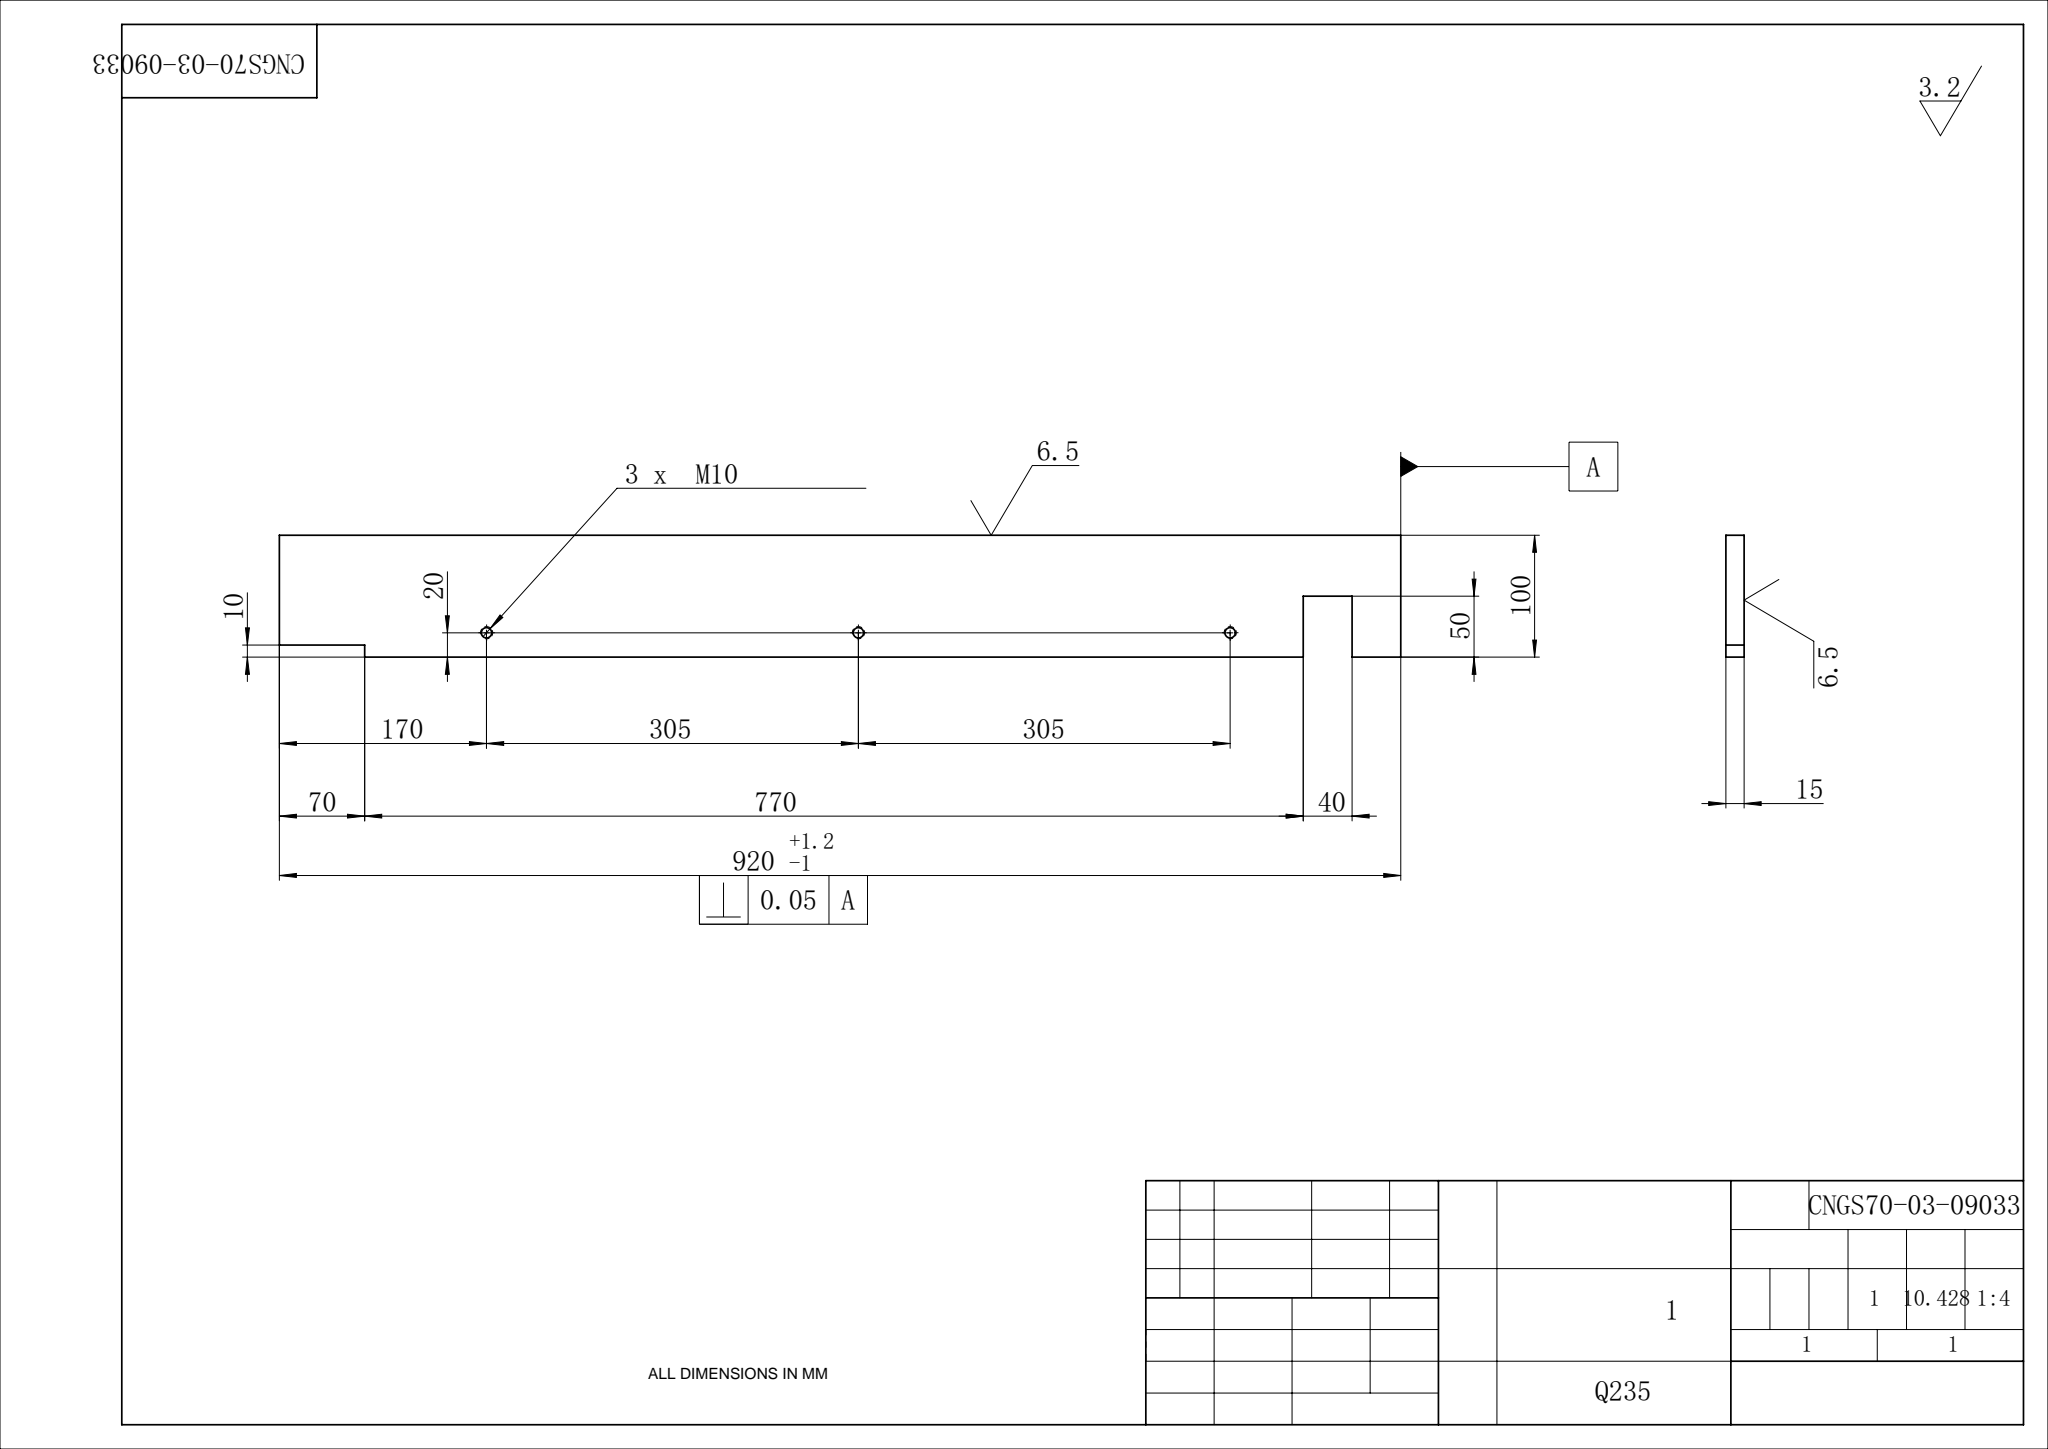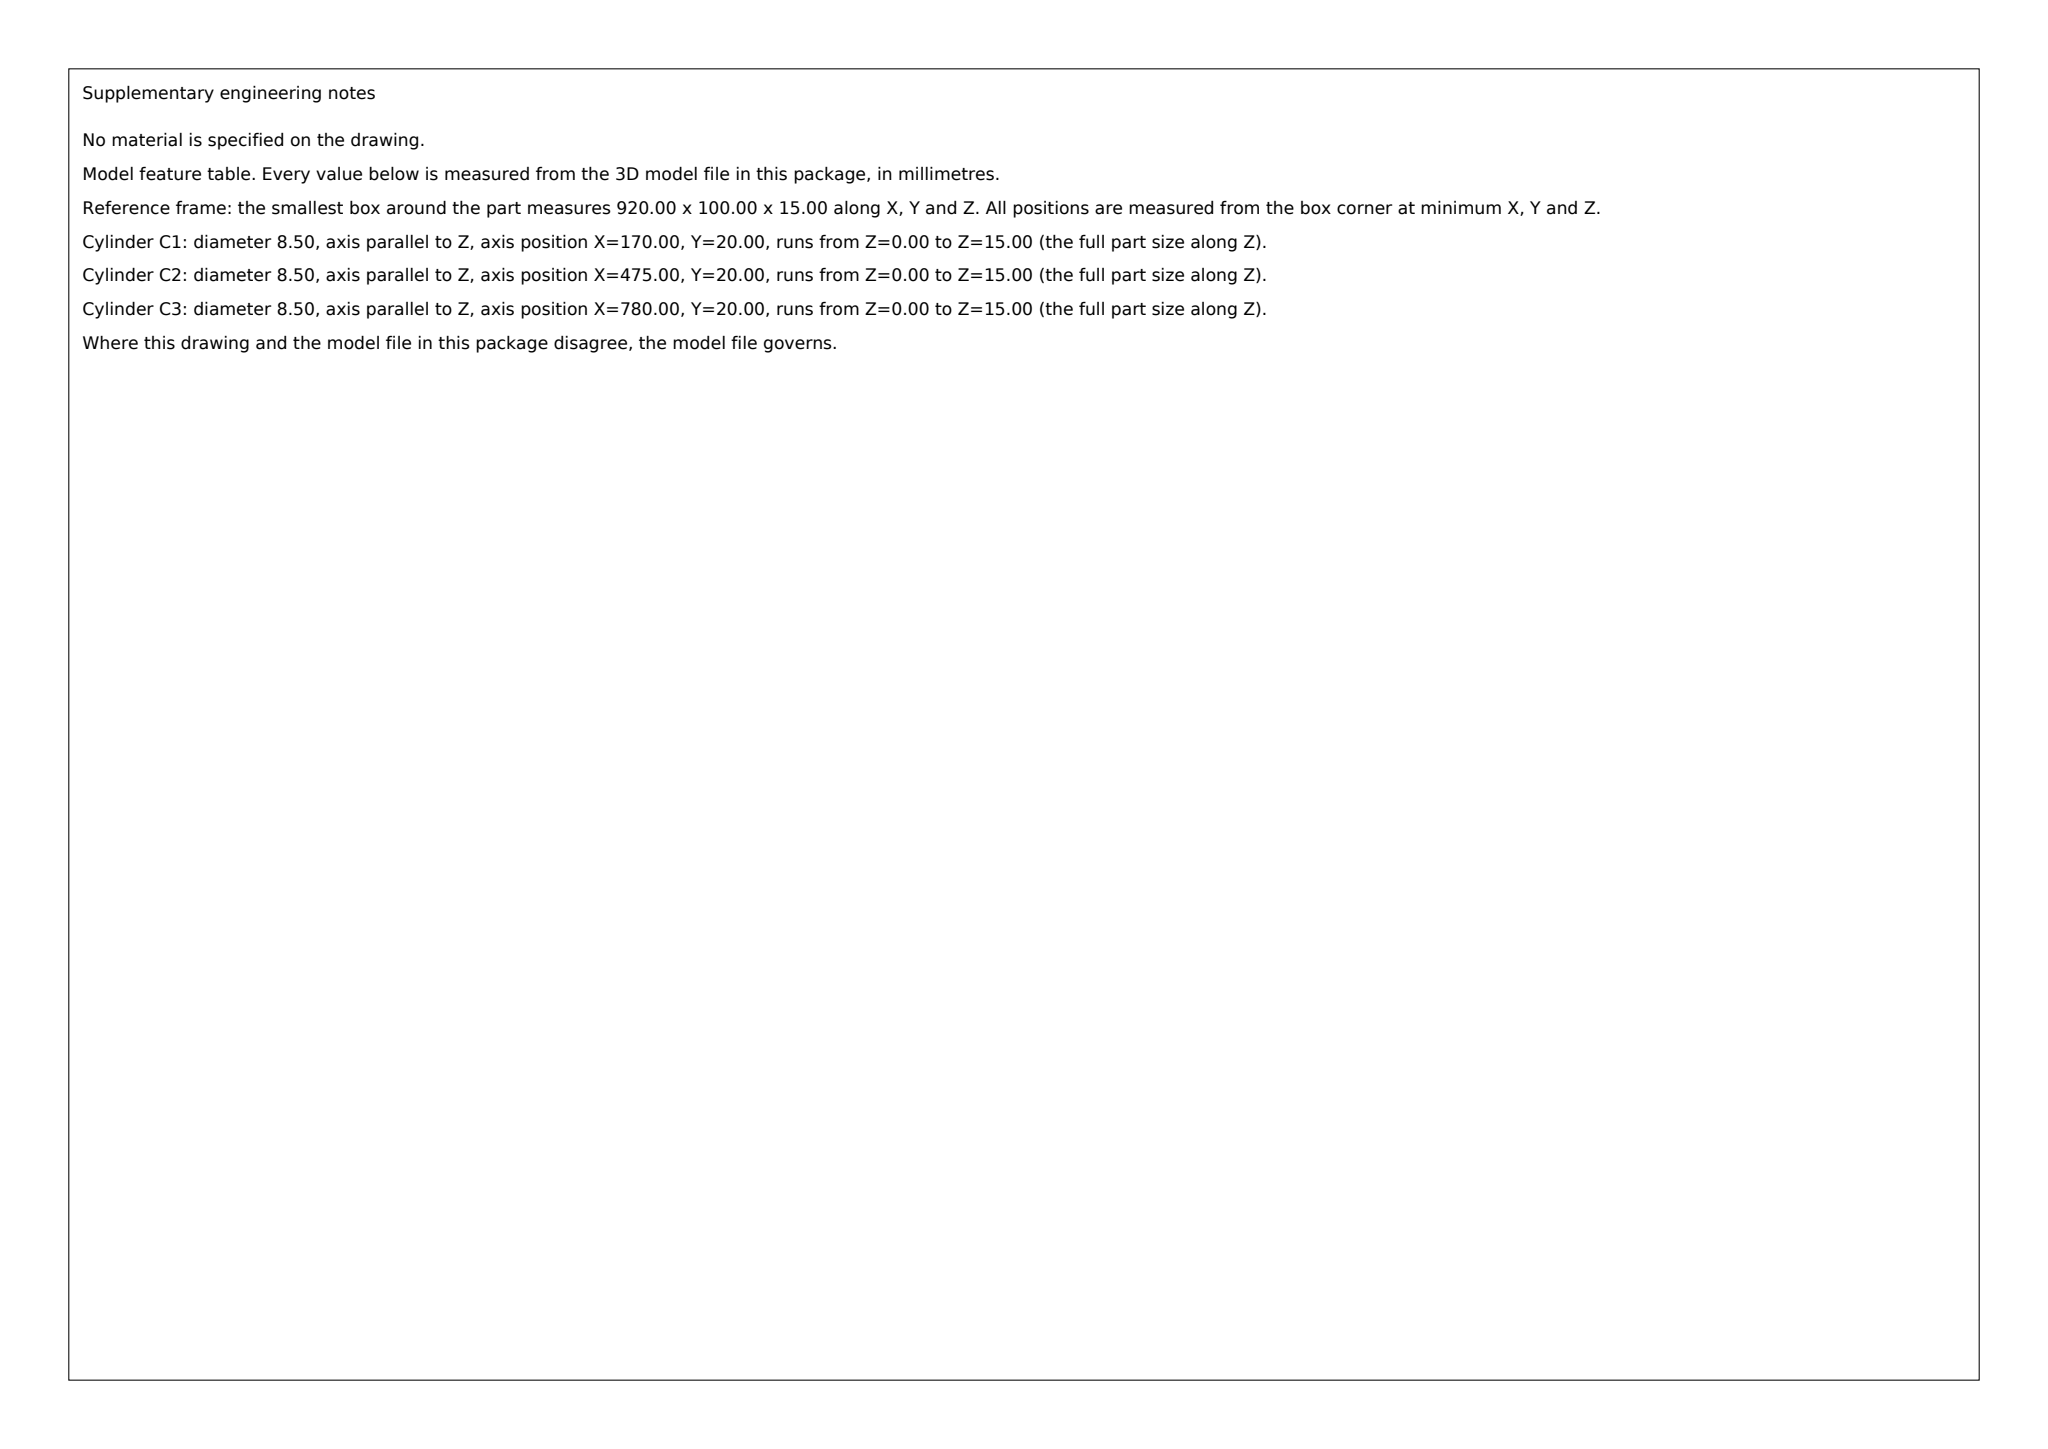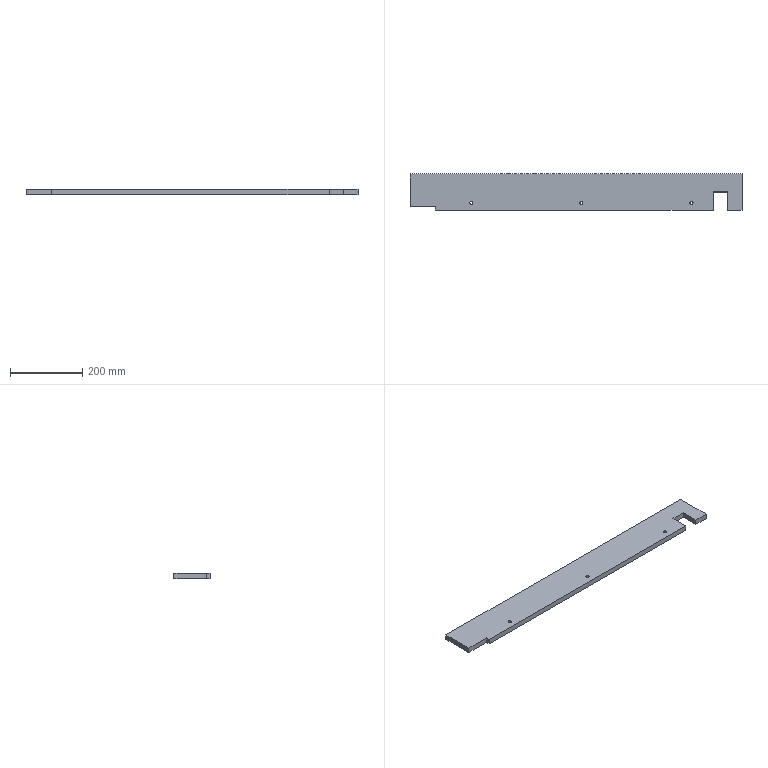Part | SolidWorks | mm | material Q235 | 1 solid | 18 faces | box 920 x 100 x 15 mm | volume 1336946 mm3 | plane 12 | cylinder 6 | commonest cylinder face diameters 8.5 x6
build123d program:
from build123d import *

# Parameters (mm, degrees)
SKETCH1_W              = 920
SKETCH1_H              = 100
BOSS_EXTRUDE1_DEPTH    = 15
M10_TAPPED_HOLE1_D     = 8.5
M10_TAPPED_HOLE1_DEPTH = 27.5
M10_TAPPED_HOLE1_TIP   = 2.554
SKETCH6_W              = 40
SKETCH6_H              = 50
SKETCH6_W_2            = 70
SKETCH6_H_2            = 10
CUT_EXTRUDE1_DEPTH     = 926.54


with BuildPart() as part:
    # Sketch1 → Boss-Extrude1 (new body)
    with BuildSketch(Plane.XY):
        with Locations((460, 50)):
            Rectangle(SKETCH1_W, SKETCH1_H)
    extrude(amount=BOSS_EXTRUDE1_DEPTH)

    # M10 Tapped Hole1
    with Locations(Plane(origin=(0, 0, 0), x_dir=(-1, 0, 0), z_dir=(0, 0, -1))):
        with Locations((-780, 20), (-475, 20), (-170, 20)):
            Hole(M10_TAPPED_HOLE1_D / 2, depth=M10_TAPPED_HOLE1_DEPTH)
            with Locations((0, 0, -(M10_TAPPED_HOLE1_DEPTH + M10_TAPPED_HOLE1_TIP / 2))):  # 118° drill point
                Cone(0, M10_TAPPED_HOLE1_D / 2, M10_TAPPED_HOLE1_TIP, mode=Mode.SUBTRACT)

    # Sketch6 → Cut-Extrude1 (cut, through all)
    with BuildSketch(Plane.XY.offset(15)):
        with Locations((860, 25)):
            Rectangle(SKETCH6_W, SKETCH6_H)
        with Locations((35, 5)):
            Rectangle(SKETCH6_W_2, SKETCH6_H_2)
    extrude(amount=-CUT_EXTRUDE1_DEPTH, mode=Mode.SUBTRACT)


solid = part.part
STEP:
#1=CARTESIAN_POINT('',(775.75,20.,15.));
#2=VERTEX_POINT('',#1);
#3=CARTESIAN_POINT('',(784.25,20.,15.));
#4=VERTEX_POINT('',#3);
#5=CARTESIAN_POINT('',(780.,20.,15.));
#6=DIRECTION('',(0.,0.,1.));
#7=DIRECTION('',(1.,0.,0.));
#8=AXIS2_PLACEMENT_3D('',#5,#6,#7);
#9=CIRCLE('',#8,4.25);
#10=EDGE_CURVE('',#2,#4,#9,.T.);
#11=ORIENTED_EDGE('',*,*,#10,.T.);
#12=CARTESIAN_POINT('',(784.25,20.,0.));
#13=VERTEX_POINT('',#12);
#14=CARTESIAN_POINT('',(784.25,20.,0.));
#15=DIRECTION('',(0.,0.,-1.));
#16=VECTOR('',#15,1000.);
#17=LINE('',#14,#16);
#18=EDGE_CURVE('',#4,#13,#17,.T.);
#19=ORIENTED_EDGE('',*,*,#18,.T.);
#20=CARTESIAN_POINT('',(775.75,20.,0.));
#21=VERTEX_POINT('',#20);
#22=CARTESIAN_POINT('',(780.,20.,0.));
#23=DIRECTION('',(0.,0.,-1.));
#24=DIRECTION('',(-1.,0.,0.));
#25=AXIS2_PLACEMENT_3D('',#22,#23,#24);
#26=CIRCLE('',#25,4.25);
#27=EDGE_CURVE('',#13,#21,#26,.T.);
#28=ORIENTED_EDGE('',*,*,#27,.T.);
#29=CARTESIAN_POINT('',(775.75,20.,0.));
#30=DIRECTION('',(0.,0.,-1.));
#31=VECTOR('',#30,1000.);
#32=LINE('',#29,#31);
#33=EDGE_CURVE('',#2,#21,#32,.T.);
#34=ORIENTED_EDGE('',*,*,#33,.F.);
#35=EDGE_LOOP('',(#11,#19,#28,#34));
#36=FACE_OUTER_BOUND('',#35,.T.);
#37=CARTESIAN_POINT('',(780.,20.,0.));
#38=DIRECTION('',(0.,0.,-1.));
#39=DIRECTION('',(-1.,0.,0.));
#40=AXIS2_PLACEMENT_3D('',#37,#38,#39);
#41=CYLINDRICAL_SURFACE('',#40,4.25);
#42=ADVANCED_FACE('',(#36),#41,.F.);
#43=CARTESIAN_POINT('',(470.75,20.,15.));
#44=VERTEX_POINT('',#43);
#45=CARTESIAN_POINT('',(479.25,20.,15.));
#46=VERTEX_POINT('',#45);
#47=CARTESIAN_POINT('',(475.,20.,15.));
#48=DIRECTION('',(0.,0.,1.));
#49=DIRECTION('',(1.,0.,0.));
#50=AXIS2_PLACEMENT_3D('',#47,#48,#49);
#51=CIRCLE('',#50,4.25);
#52=EDGE_CURVE('',#44,#46,#51,.T.);
#53=ORIENTED_EDGE('',*,*,#52,.T.);
#54=CARTESIAN_POINT('',(479.25,20.,0.));
#55=VERTEX_POINT('',#54);
#56=CARTESIAN_POINT('',(479.25,20.,0.));
#57=DIRECTION('',(0.,0.,-1.));
#58=VECTOR('',#57,1000.);
#59=LINE('',#56,#58);
#60=EDGE_CURVE('',#46,#55,#59,.T.);
#61=ORIENTED_EDGE('',*,*,#60,.T.);
#62=CARTESIAN_POINT('',(470.75,20.,0.));
#63=VERTEX_POINT('',#62);
#64=CARTESIAN_POINT('',(475.,20.,0.));
#65=DIRECTION('',(0.,0.,-1.));
#66=DIRECTION('',(-1.,0.,0.));
#67=AXIS2_PLACEMENT_3D('',#64,#65,#66);
#68=CIRCLE('',#67,4.25);
#69=EDGE_CURVE('',#55,#63,#68,.T.);
#70=ORIENTED_EDGE('',*,*,#69,.T.);
#71=CARTESIAN_POINT('',(470.75,20.,0.));
#72=DIRECTION('',(0.,0.,-1.));
#73=VECTOR('',#72,1000.);
#74=LINE('',#71,#73);
#75=EDGE_CURVE('',#44,#63,#74,.T.);
#76=ORIENTED_EDGE('',*,*,#75,.F.);
#77=EDGE_LOOP('',(#53,#61,#70,#76));
#78=FACE_OUTER_BOUND('',#77,.T.);
#79=CARTESIAN_POINT('',(475.,20.,0.));
#80=DIRECTION('',(0.,0.,-1.));
#81=DIRECTION('',(-1.,0.,0.));
#82=AXIS2_PLACEMENT_3D('',#79,#80,#81);
#83=CYLINDRICAL_SURFACE('',#82,4.25);
#84=ADVANCED_FACE('',(#78),#83,.F.);
#85=CARTESIAN_POINT('',(165.75,20.,15.));
#86=VERTEX_POINT('',#85);
#87=CARTESIAN_POINT('',(174.25,20.,15.));
#88=VERTEX_POINT('',#87);
#89=CARTESIAN_POINT('',(170.,20.,15.));
#90=DIRECTION('',(0.,0.,1.));
#91=DIRECTION('',(1.,0.,0.));
#92=AXIS2_PLACEMENT_3D('',#89,#90,#91);
#93=CIRCLE('',#92,4.25);
#94=EDGE_CURVE('',#86,#88,#93,.T.);
#95=ORIENTED_EDGE('',*,*,#94,.T.);
#96=CARTESIAN_POINT('',(174.25,20.,0.));
#97=VERTEX_POINT('',#96);
#98=CARTESIAN_POINT('',(174.25,20.,0.));
#99=DIRECTION('',(0.,0.,-1.));
#100=VECTOR('',#99,1000.);
#101=LINE('',#98,#100);
#102=EDGE_CURVE('',#88,#97,#101,.T.);
#103=ORIENTED_EDGE('',*,*,#102,.T.);
#104=CARTESIAN_POINT('',(165.75,20.,0.));
#105=VERTEX_POINT('',#104);
#106=CARTESIAN_POINT('',(170.,20.,0.));
#107=DIRECTION('',(0.,0.,-1.));
#108=DIRECTION('',(-1.,0.,0.));
#109=AXIS2_PLACEMENT_3D('',#106,#107,#108);
#110=CIRCLE('',#109,4.25);
#111=EDGE_CURVE('',#97,#105,#110,.T.);
#112=ORIENTED_EDGE('',*,*,#111,.T.);
#113=CARTESIAN_POINT('',(165.75,20.,0.));
#114=DIRECTION('',(0.,0.,-1.));
#115=VECTOR('',#114,1000.);
#116=LINE('',#113,#115);
#117=EDGE_CURVE('',#86,#105,#116,.T.);
#118=ORIENTED_EDGE('',*,*,#117,.F.);
#119=EDGE_LOOP('',(#95,#103,#112,#118));
#120=FACE_OUTER_BOUND('',#119,.T.);
#121=CARTESIAN_POINT('',(170.,20.,0.));
#122=DIRECTION('',(0.,0.,-1.));
#123=DIRECTION('',(-1.,0.,0.));
#124=AXIS2_PLACEMENT_3D('',#121,#122,#123);
#125=CYLINDRICAL_SURFACE('',#124,4.25);
#126=ADVANCED_FACE('',(#120),#125,.F.);
#127=CARTESIAN_POINT('',(70.,0.,15.));
#128=VERTEX_POINT('',#127);
#129=CARTESIAN_POINT('',(840.,0.,15.));
#130=VERTEX_POINT('',#129);
#131=CARTESIAN_POINT('',(0.,0.,15.));
#132=DIRECTION('',(1.,0.,0.));
#133=VECTOR('',#132,1000.);
#134=LINE('',#131,#133);
#135=EDGE_CURVE('',#128,#130,#134,.T.);
#136=ORIENTED_EDGE('',*,*,#135,.F.);
#137=CARTESIAN_POINT('',(70.,0.,0.));
#138=VERTEX_POINT('',#137);
#139=CARTESIAN_POINT('',(70.,0.,0.));
#140=DIRECTION('',(0.,0.,1.));
#141=VECTOR('',#140,1000.);
#142=LINE('',#139,#141);
#143=EDGE_CURVE('',#138,#128,#142,.T.);
#144=ORIENTED_EDGE('',*,*,#143,.F.);
#145=CARTESIAN_POINT('',(840.,0.,0.));
#146=VERTEX_POINT('',#145);
#147=CARTESIAN_POINT('',(0.,0.,0.));
#148=DIRECTION('',(1.,0.,0.));
#149=VECTOR('',#148,1000.);
#150=LINE('',#147,#149);
#151=EDGE_CURVE('',#138,#146,#150,.T.);
#152=ORIENTED_EDGE('',*,*,#151,.T.);
#153=CARTESIAN_POINT('',(840.,0.,0.));
#154=DIRECTION('',(0.,0.,1.));
#155=VECTOR('',#154,1000.);
#156=LINE('',#153,#155);
#157=EDGE_CURVE('',#146,#130,#156,.T.);
#158=ORIENTED_EDGE('',*,*,#157,.T.);
#159=EDGE_LOOP('',(#136,#144,#152,#158));
#160=FACE_OUTER_BOUND('',#159,.T.);
#161=CARTESIAN_POINT('',(0.,0.,15.));
#162=DIRECTION('',(0.,1.,0.));
#163=DIRECTION('',(0.,0.,1.));
#164=AXIS2_PLACEMENT_3D('',#161,#162,#163);
#165=PLANE('',#164);
#166=ADVANCED_FACE('',(#160),#165,.F.);
#167=CARTESIAN_POINT('',(920.,100.,0.));
#168=VERTEX_POINT('',#167);
#169=CARTESIAN_POINT('',(920.,0.,0.));
#170=VERTEX_POINT('',#169);
#171=CARTESIAN_POINT('',(920.,0.,0.));
#172=DIRECTION('',(0.,-1.,0.));
#173=VECTOR('',#172,1000.);
#174=LINE('',#171,#173);
#175=EDGE_CURVE('',#168,#170,#174,.T.);
#176=ORIENTED_EDGE('',*,*,#175,.F.);
#177=CARTESIAN_POINT('',(920.,100.,15.));
#178=VERTEX_POINT('',#177);
#179=CARTESIAN_POINT('',(920.,100.,15.));
#180=DIRECTION('',(0.,0.,-1.));
#181=VECTOR('',#180,1000.);
#182=LINE('',#179,#181);
#183=EDGE_CURVE('',#178,#168,#182,.T.);
#184=ORIENTED_EDGE('',*,*,#183,.F.);
#185=CARTESIAN_POINT('',(920.,0.,15.));
#186=VERTEX_POINT('',#185);
#187=CARTESIAN_POINT('',(920.,0.,15.));
#188=DIRECTION('',(0.,-1.,0.));
#189=VECTOR('',#188,1000.);
#190=LINE('',#187,#189);
#191=EDGE_CURVE('',#178,#186,#190,.T.);
#192=ORIENTED_EDGE('',*,*,#191,.T.);
#193=CARTESIAN_POINT('',(920.,0.,15.));
#194=DIRECTION('',(0.,0.,-1.));
#195=VECTOR('',#194,1000.);
#196=LINE('',#193,#195);
#197=EDGE_CURVE('',#186,#170,#196,.T.);
#198=ORIENTED_EDGE('',*,*,#197,.T.);
#199=EDGE_LOOP('',(#176,#184,#192,#198));
#200=FACE_OUTER_BOUND('',#199,.T.);
#201=CARTESIAN_POINT('',(920.,0.,15.));
#202=DIRECTION('',(1.,0.,0.));
#203=DIRECTION('',(0.,0.,-1.));
#204=AXIS2_PLACEMENT_3D('',#201,#202,#203);
#205=PLANE('',#204);
#206=ADVANCED_FACE('',(#200),#205,.T.);
#207=CARTESIAN_POINT('',(0.,100.,0.));
#208=VERTEX_POINT('',#207);
#209=CARTESIAN_POINT('',(0.,100.,0.));
#210=DIRECTION('',(1.,-0.,0.));
#211=VECTOR('',#210,1000.);
#212=LINE('',#209,#211);
#213=EDGE_CURVE('',#208,#168,#212,.T.);
#214=ORIENTED_EDGE('',*,*,#213,.F.);
#215=CARTESIAN_POINT('',(0.,100.,15.));
#216=VERTEX_POINT('',#215);
#217=CARTESIAN_POINT('',(0.,100.,15.));
#218=DIRECTION('',(0.,0.,-1.));
#219=VECTOR('',#218,1000.);
#220=LINE('',#217,#219);
#221=EDGE_CURVE('',#216,#208,#220,.T.);
#222=ORIENTED_EDGE('',*,*,#221,.F.);
#223=CARTESIAN_POINT('',(0.,100.,15.));
#224=DIRECTION('',(1.,-0.,0.));
#225=VECTOR('',#224,1000.);
#226=LINE('',#223,#225);
#227=EDGE_CURVE('',#216,#178,#226,.T.);
#228=ORIENTED_EDGE('',*,*,#227,.T.);
#229=ORIENTED_EDGE('',*,*,#183,.T.);
#230=EDGE_LOOP('',(#214,#222,#228,#229));
#231=FACE_OUTER_BOUND('',#230,.T.);
#232=CARTESIAN_POINT('',(0.,100.,15.));
#233=DIRECTION('',(0.,1.,0.));
#234=DIRECTION('',(-1.,0.,0.));
#235=AXIS2_PLACEMENT_3D('',#232,#233,#234);
#236=PLANE('',#235);
#237=ADVANCED_FACE('',(#231),#236,.T.);
#238=CARTESIAN_POINT('',(0.,10.,0.));
#239=VERTEX_POINT('',#238);
#240=CARTESIAN_POINT('',(0.,10.,15.));
#241=VERTEX_POINT('',#240);
#242=CARTESIAN_POINT('',(0.,10.,0.));
#243=DIRECTION('',(0.,0.,1.));
#244=VECTOR('',#243,1000.);
#245=LINE('',#242,#244);
#246=EDGE_CURVE('',#239,#241,#245,.T.);
#247=ORIENTED_EDGE('',*,*,#246,.T.);
#248=CARTESIAN_POINT('',(0.,0.,15.));
#249=DIRECTION('',(0.,1.,0.));
#250=VECTOR('',#249,1000.);
#251=LINE('',#248,#250);
#252=EDGE_CURVE('',#241,#216,#251,.T.);
#253=ORIENTED_EDGE('',*,*,#252,.T.);
#254=ORIENTED_EDGE('',*,*,#221,.T.);
#255=CARTESIAN_POINT('',(0.,0.,0.));
#256=DIRECTION('',(0.,1.,0.));
#257=VECTOR('',#256,1000.);
#258=LINE('',#255,#257);
#259=EDGE_CURVE('',#239,#208,#258,.T.);
#260=ORIENTED_EDGE('',*,*,#259,.F.);
#261=EDGE_LOOP('',(#247,#253,#254,#260));
#262=FACE_OUTER_BOUND('',#261,.T.);
#263=CARTESIAN_POINT('',(0.,0.,15.));
#264=DIRECTION('',(-1.,0.,0.));
#265=DIRECTION('',(0.,0.,1.));
#266=AXIS2_PLACEMENT_3D('',#263,#264,#265);
#267=PLANE('',#266);
#268=ADVANCED_FACE('',(#262),#267,.T.);
#269=CARTESIAN_POINT('',(880.,0.,15.));
#270=VERTEX_POINT('',#269);
#271=CARTESIAN_POINT('',(0.,0.,15.));
#272=DIRECTION('',(1.,0.,0.));
#273=VECTOR('',#272,1000.);
#274=LINE('',#271,#273);
#275=EDGE_CURVE('',#270,#186,#274,.T.);
#276=ORIENTED_EDGE('',*,*,#275,.F.);
#277=CARTESIAN_POINT('',(880.,0.,0.));
#278=VERTEX_POINT('',#277);
#279=CARTESIAN_POINT('',(880.,0.,0.));
#280=DIRECTION('',(0.,0.,1.));
#281=VECTOR('',#280,1000.);
#282=LINE('',#279,#281);
#283=EDGE_CURVE('',#278,#270,#282,.T.);
#284=ORIENTED_EDGE('',*,*,#283,.F.);
#285=CARTESIAN_POINT('',(0.,0.,0.));
#286=DIRECTION('',(1.,0.,0.));
#287=VECTOR('',#286,1000.);
#288=LINE('',#285,#287);
#289=EDGE_CURVE('',#278,#170,#288,.T.);
#290=ORIENTED_EDGE('',*,*,#289,.T.);
#291=ORIENTED_EDGE('',*,*,#197,.F.);
#292=EDGE_LOOP('',(#276,#284,#290,#291));
#293=FACE_OUTER_BOUND('',#292,.T.);
#294=CARTESIAN_POINT('',(0.,0.,15.));
#295=DIRECTION('',(0.,1.,0.));
#296=DIRECTION('',(0.,0.,1.));
#297=AXIS2_PLACEMENT_3D('',#294,#295,#296);
#298=PLANE('',#297);
#299=ADVANCED_FACE('',(#293),#298,.F.);
#300=CARTESIAN_POINT('',(70.,10.,15.));
#301=VERTEX_POINT('',#300);
#302=CARTESIAN_POINT('',(0.,10.,15.));
#303=DIRECTION('',(-1.,0.,0.));
#304=VECTOR('',#303,1000.);
#305=LINE('',#302,#304);
#306=EDGE_CURVE('',#301,#241,#305,.T.);
#307=ORIENTED_EDGE('',*,*,#306,.F.);
#308=CARTESIAN_POINT('',(70.,0.,15.));
#309=DIRECTION('',(0.,1.,0.));
#310=VECTOR('',#309,1000.);
#311=LINE('',#308,#310);
#312=EDGE_CURVE('',#128,#301,#311,.T.);
#313=ORIENTED_EDGE('',*,*,#312,.F.);
#314=ORIENTED_EDGE('',*,*,#135,.T.);
#315=CARTESIAN_POINT('',(840.,50.,15.));
#316=VERTEX_POINT('',#315);
#317=CARTESIAN_POINT('',(840.,0.,15.));
#318=DIRECTION('',(0.,-1.,0.));
#319=VECTOR('',#318,1000.);
#320=LINE('',#317,#319);
#321=EDGE_CURVE('',#316,#130,#320,.T.);
#322=ORIENTED_EDGE('',*,*,#321,.F.);
#323=CARTESIAN_POINT('',(880.,50.,15.));
#324=VERTEX_POINT('',#323);
#325=CARTESIAN_POINT('',(840.,50.,15.));
#326=DIRECTION('',(-1.,0.,0.));
#327=VECTOR('',#326,1000.);
#328=LINE('',#325,#327);
#329=EDGE_CURVE('',#324,#316,#328,.T.);
#330=ORIENTED_EDGE('',*,*,#329,.F.);
#331=CARTESIAN_POINT('',(880.,0.,15.));
#332=DIRECTION('',(0.,1.,0.));
#333=VECTOR('',#332,1000.);
#334=LINE('',#331,#333);
#335=EDGE_CURVE('',#270,#324,#334,.T.);
#336=ORIENTED_EDGE('',*,*,#335,.F.);
#337=ORIENTED_EDGE('',*,*,#275,.T.);
#338=ORIENTED_EDGE('',*,*,#191,.F.);
#339=ORIENTED_EDGE('',*,*,#227,.F.);
#340=ORIENTED_EDGE('',*,*,#252,.F.);
#341=EDGE_LOOP('',(#307,#313,#314,#322,#330,#336,#337,#338,#339,#340));
#342=FACE_OUTER_BOUND('',#341,.T.);
#343=ORIENTED_EDGE('',*,*,#10,.F.);
#344=CARTESIAN_POINT('',(780.,20.,15.));
#345=DIRECTION('',(0.,0.,1.));
#346=DIRECTION('',(1.,0.,0.));
#347=AXIS2_PLACEMENT_3D('',#344,#345,#346);
#348=CIRCLE('',#347,4.25);
#349=EDGE_CURVE('',#4,#2,#348,.T.);
#350=ORIENTED_EDGE('',*,*,#349,.F.);
#351=EDGE_LOOP('',(#343,#350));
#352=FACE_BOUND('',#351,.T.);
#353=ORIENTED_EDGE('',*,*,#52,.F.);
#354=CARTESIAN_POINT('',(475.,20.,15.));
#355=DIRECTION('',(0.,0.,1.));
#356=DIRECTION('',(1.,0.,0.));
#357=AXIS2_PLACEMENT_3D('',#354,#355,#356);
#358=CIRCLE('',#357,4.25);
#359=EDGE_CURVE('',#46,#44,#358,.T.);
#360=ORIENTED_EDGE('',*,*,#359,.F.);
#361=EDGE_LOOP('',(#353,#360));
#362=FACE_BOUND('',#361,.T.);
#363=ORIENTED_EDGE('',*,*,#94,.F.);
#364=CARTESIAN_POINT('',(170.,20.,15.));
#365=DIRECTION('',(0.,0.,1.));
#366=DIRECTION('',(1.,0.,0.));
#367=AXIS2_PLACEMENT_3D('',#364,#365,#366);
#368=CIRCLE('',#367,4.25);
#369=EDGE_CURVE('',#88,#86,#368,.T.);
#370=ORIENTED_EDGE('',*,*,#369,.F.);
#371=EDGE_LOOP('',(#363,#370));
#372=FACE_BOUND('',#371,.T.);
#373=CARTESIAN_POINT('',(0.,0.,15.));
#374=DIRECTION('',(0.,0.,1.));
#375=DIRECTION('',(1.,0.,0.));
#376=AXIS2_PLACEMENT_3D('',#373,#374,#375);
#377=PLANE('',#376);
#378=ADVANCED_FACE('',(#342,#352,#362,#372),#377,.T.);
#379=CARTESIAN_POINT('',(780.,20.,0.));
#380=DIRECTION('',(0.,0.,-1.));
#381=DIRECTION('',(-1.,0.,0.));
#382=AXIS2_PLACEMENT_3D('',#379,#380,#381);
#383=CIRCLE('',#382,4.25);
#384=EDGE_CURVE('',#21,#13,#383,.T.);
#385=ORIENTED_EDGE('',*,*,#384,.F.);
#386=ORIENTED_EDGE('',*,*,#27,.F.);
#387=EDGE_LOOP('',(#385,#386));
#388=FACE_BOUND('',#387,.T.);
#389=CARTESIAN_POINT('',(475.,20.,0.));
#390=DIRECTION('',(0.,0.,-1.));
#391=DIRECTION('',(-1.,0.,0.));
#392=AXIS2_PLACEMENT_3D('',#389,#390,#391);
#393=CIRCLE('',#392,4.25);
#394=EDGE_CURVE('',#63,#55,#393,.T.);
#395=ORIENTED_EDGE('',*,*,#394,.F.);
#396=ORIENTED_EDGE('',*,*,#69,.F.);
#397=EDGE_LOOP('',(#395,#396));
#398=FACE_BOUND('',#397,.T.);
#399=CARTESIAN_POINT('',(170.,20.,0.));
#400=DIRECTION('',(0.,0.,-1.));
#401=DIRECTION('',(-1.,0.,0.));
#402=AXIS2_PLACEMENT_3D('',#399,#400,#401);
#403=CIRCLE('',#402,4.25);
#404=EDGE_CURVE('',#105,#97,#403,.T.);
#405=ORIENTED_EDGE('',*,*,#404,.F.);
#406=ORIENTED_EDGE('',*,*,#111,.F.);
#407=EDGE_LOOP('',(#405,#406));
#408=FACE_BOUND('',#407,.T.);
#409=CARTESIAN_POINT('',(70.,10.,0.));
#410=VERTEX_POINT('',#409);
#411=CARTESIAN_POINT('',(70.,0.,0.));
#412=DIRECTION('',(0.,1.,0.));
#413=VECTOR('',#412,1000.);
#414=LINE('',#411,#413);
#415=EDGE_CURVE('',#138,#410,#414,.T.);
#416=ORIENTED_EDGE('',*,*,#415,.T.);
#417=CARTESIAN_POINT('',(0.,10.,0.));
#418=DIRECTION('',(-1.,0.,0.));
#419=VECTOR('',#418,1000.);
#420=LINE('',#417,#419);
#421=EDGE_CURVE('',#410,#239,#420,.T.);
#422=ORIENTED_EDGE('',*,*,#421,.T.);
#423=ORIENTED_EDGE('',*,*,#259,.T.);
#424=ORIENTED_EDGE('',*,*,#213,.T.);
#425=ORIENTED_EDGE('',*,*,#175,.T.);
#426=ORIENTED_EDGE('',*,*,#289,.F.);
#427=CARTESIAN_POINT('',(880.,50.,0.));
#428=VERTEX_POINT('',#427);
#429=CARTESIAN_POINT('',(880.,0.,0.));
#430=DIRECTION('',(0.,1.,0.));
#431=VECTOR('',#430,1000.);
#432=LINE('',#429,#431);
#433=EDGE_CURVE('',#278,#428,#432,.T.);
#434=ORIENTED_EDGE('',*,*,#433,.T.);
#435=CARTESIAN_POINT('',(840.,50.,0.));
#436=VERTEX_POINT('',#435);
#437=CARTESIAN_POINT('',(840.,50.,0.));
#438=DIRECTION('',(-1.,0.,0.));
#439=VECTOR('',#438,1000.);
#440=LINE('',#437,#439);
#441=EDGE_CURVE('',#428,#436,#440,.T.);
#442=ORIENTED_EDGE('',*,*,#441,.T.);
#443=CARTESIAN_POINT('',(840.,0.,0.));
#444=DIRECTION('',(0.,-1.,0.));
#445=VECTOR('',#444,1000.);
#446=LINE('',#443,#445);
#447=EDGE_CURVE('',#436,#146,#446,.T.);
#448=ORIENTED_EDGE('',*,*,#447,.T.);
#449=ORIENTED_EDGE('',*,*,#151,.F.);
#450=EDGE_LOOP('',(#416,#422,#423,#424,#425,#426,#434,#442,#448,#449));
#451=FACE_OUTER_BOUND('',#450,.T.);
#452=CARTESIAN_POINT('',(0.,0.,0.));
#453=DIRECTION('',(0.,0.,1.));
#454=DIRECTION('',(1.,0.,0.));
#455=AXIS2_PLACEMENT_3D('',#452,#453,#454);
#456=PLANE('',#455);
#457=ADVANCED_FACE('',(#388,#398,#408,#451),#456,.F.);
#458=ORIENTED_EDGE('',*,*,#102,.F.);
#459=ORIENTED_EDGE('',*,*,#369,.T.);
#460=ORIENTED_EDGE('',*,*,#117,.T.);
#461=ORIENTED_EDGE('',*,*,#404,.T.);
#462=EDGE_LOOP('',(#458,#459,#460,#461));
#463=FACE_OUTER_BOUND('',#462,.T.);
#464=CARTESIAN_POINT('',(170.,20.,0.));
#465=DIRECTION('',(0.,0.,-1.));
#466=DIRECTION('',(-1.,0.,0.));
#467=AXIS2_PLACEMENT_3D('',#464,#465,#466);
#468=CYLINDRICAL_SURFACE('',#467,4.25);
#469=ADVANCED_FACE('',(#463),#468,.F.);
#470=ORIENTED_EDGE('',*,*,#60,.F.);
#471=ORIENTED_EDGE('',*,*,#359,.T.);
#472=ORIENTED_EDGE('',*,*,#75,.T.);
#473=ORIENTED_EDGE('',*,*,#394,.T.);
#474=EDGE_LOOP('',(#470,#471,#472,#473));
#475=FACE_OUTER_BOUND('',#474,.T.);
#476=CARTESIAN_POINT('',(475.,20.,0.));
#477=DIRECTION('',(0.,0.,-1.));
#478=DIRECTION('',(-1.,0.,0.));
#479=AXIS2_PLACEMENT_3D('',#476,#477,#478);
#480=CYLINDRICAL_SURFACE('',#479,4.25);
#481=ADVANCED_FACE('',(#475),#480,.F.);
#482=ORIENTED_EDGE('',*,*,#18,.F.);
#483=ORIENTED_EDGE('',*,*,#349,.T.);
#484=ORIENTED_EDGE('',*,*,#33,.T.);
#485=ORIENTED_EDGE('',*,*,#384,.T.);
#486=EDGE_LOOP('',(#482,#483,#484,#485));
#487=FACE_OUTER_BOUND('',#486,.T.);
#488=CARTESIAN_POINT('',(780.,20.,0.));
#489=DIRECTION('',(0.,0.,-1.));
#490=DIRECTION('',(-1.,0.,0.));
#491=AXIS2_PLACEMENT_3D('',#488,#489,#490);
#492=CYLINDRICAL_SURFACE('',#491,4.25);
#493=ADVANCED_FACE('',(#487),#492,.F.);
#494=ORIENTED_EDGE('',*,*,#321,.T.);
#495=ORIENTED_EDGE('',*,*,#157,.F.);
#496=ORIENTED_EDGE('',*,*,#447,.F.);
#497=CARTESIAN_POINT('',(840.,50.,0.));
#498=DIRECTION('',(0.,0.,1.));
#499=VECTOR('',#498,1000.);
#500=LINE('',#497,#499);
#501=EDGE_CURVE('',#436,#316,#500,.T.);
#502=ORIENTED_EDGE('',*,*,#501,.T.);
#503=EDGE_LOOP('',(#494,#495,#496,#502));
#504=FACE_OUTER_BOUND('',#503,.T.);
#505=CARTESIAN_POINT('',(840.,0.,0.));
#506=DIRECTION('',(-1.,0.,0.));
#507=DIRECTION('',(0.,0.,1.));
#508=AXIS2_PLACEMENT_3D('',#505,#506,#507);
#509=PLANE('',#508);
#510=ADVANCED_FACE('',(#504),#509,.F.);
#511=ORIENTED_EDGE('',*,*,#329,.T.);
#512=ORIENTED_EDGE('',*,*,#501,.F.);
#513=ORIENTED_EDGE('',*,*,#441,.F.);
#514=CARTESIAN_POINT('',(880.,50.,0.));
#515=DIRECTION('',(0.,0.,1.));
#516=VECTOR('',#515,1000.);
#517=LINE('',#514,#516);
#518=EDGE_CURVE('',#428,#324,#517,.T.);
#519=ORIENTED_EDGE('',*,*,#518,.T.);
#520=EDGE_LOOP('',(#511,#512,#513,#519));
#521=FACE_OUTER_BOUND('',#520,.T.);
#522=CARTESIAN_POINT('',(840.,50.,0.));
#523=DIRECTION('',(0.,1.,0.));
#524=DIRECTION('',(0.,0.,1.));
#525=AXIS2_PLACEMENT_3D('',#522,#523,#524);
#526=PLANE('',#525);
#527=ADVANCED_FACE('',(#521),#526,.F.);
#528=ORIENTED_EDGE('',*,*,#335,.T.);
#529=ORIENTED_EDGE('',*,*,#518,.F.);
#530=ORIENTED_EDGE('',*,*,#433,.F.);
#531=ORIENTED_EDGE('',*,*,#283,.T.);
#532=EDGE_LOOP('',(#528,#529,#530,#531));
#533=FACE_OUTER_BOUND('',#532,.T.);
#534=CARTESIAN_POINT('',(880.,0.,0.));
#535=DIRECTION('',(1.,0.,0.));
#536=DIRECTION('',(0.,0.,-1.));
#537=AXIS2_PLACEMENT_3D('',#534,#535,#536);
#538=PLANE('',#537);
#539=ADVANCED_FACE('',(#533),#538,.F.);
#540=ORIENTED_EDGE('',*,*,#306,.T.);
#541=ORIENTED_EDGE('',*,*,#246,.F.);
#542=ORIENTED_EDGE('',*,*,#421,.F.);
#543=CARTESIAN_POINT('',(70.,10.,0.));
#544=DIRECTION('',(0.,0.,1.));
#545=VECTOR('',#544,1000.);
#546=LINE('',#543,#545);
#547=EDGE_CURVE('',#410,#301,#546,.T.);
#548=ORIENTED_EDGE('',*,*,#547,.T.);
#549=EDGE_LOOP('',(#540,#541,#542,#548));
#550=FACE_OUTER_BOUND('',#549,.T.);
#551=CARTESIAN_POINT('',(0.,10.,0.));
#552=DIRECTION('',(0.,1.,0.));
#553=DIRECTION('',(0.,0.,1.));
#554=AXIS2_PLACEMENT_3D('',#551,#552,#553);
#555=PLANE('',#554);
#556=ADVANCED_FACE('',(#550),#555,.F.);
#557=ORIENTED_EDGE('',*,*,#312,.T.);
#558=ORIENTED_EDGE('',*,*,#547,.F.);
#559=ORIENTED_EDGE('',*,*,#415,.F.);
#560=ORIENTED_EDGE('',*,*,#143,.T.);
#561=EDGE_LOOP('',(#557,#558,#559,#560));
#562=FACE_OUTER_BOUND('',#561,.T.);
#563=CARTESIAN_POINT('',(70.,0.,0.));
#564=DIRECTION('',(1.,0.,0.));
#565=DIRECTION('',(0.,0.,-1.));
#566=AXIS2_PLACEMENT_3D('',#563,#564,#565);
#567=PLANE('',#566);
#568=ADVANCED_FACE('',(#562),#567,.F.);
#569=CLOSED_SHELL('',(#42,#84,#126,#166,#206,#237,#268,#299,#378,#457,#469,#481,#493,#510,#527,#539,#556,#568));
#570=MANIFOLD_SOLID_BREP('',#569);
#571=CARTESIAN_POINT('',(0.,0.,0.));
#572=DIRECTION('',(0.,0.,1.));
#573=DIRECTION('',(1.,0.,0.));
#574=AXIS2_PLACEMENT_3D('',#571,#572,#573);
#575=(LENGTH_UNIT()NAMED_UNIT(*)SI_UNIT(.MILLI.,.METRE.));
#576=UNCERTAINTY_MEASURE_WITH_UNIT(LENGTH_MEASURE(0.00001),#575,'','');
#577=(NAMED_UNIT(*)PLANE_ANGLE_UNIT()SI_UNIT($,.RADIAN.));
#578=(NAMED_UNIT(*)SI_UNIT($,.STERADIAN.)SOLID_ANGLE_UNIT());
#579=(GEOMETRIC_REPRESENTATION_CONTEXT(3)GLOBAL_UNCERTAINTY_ASSIGNED_CONTEXT((#576))GLOBAL_UNIT_ASSIGNED_CONTEXT((#575,#577,#578))REPRESENTATION_CONTEXT('',''));
#580=ADVANCED_BREP_SHAPE_REPRESENTATION('',(#570,#574),#579);